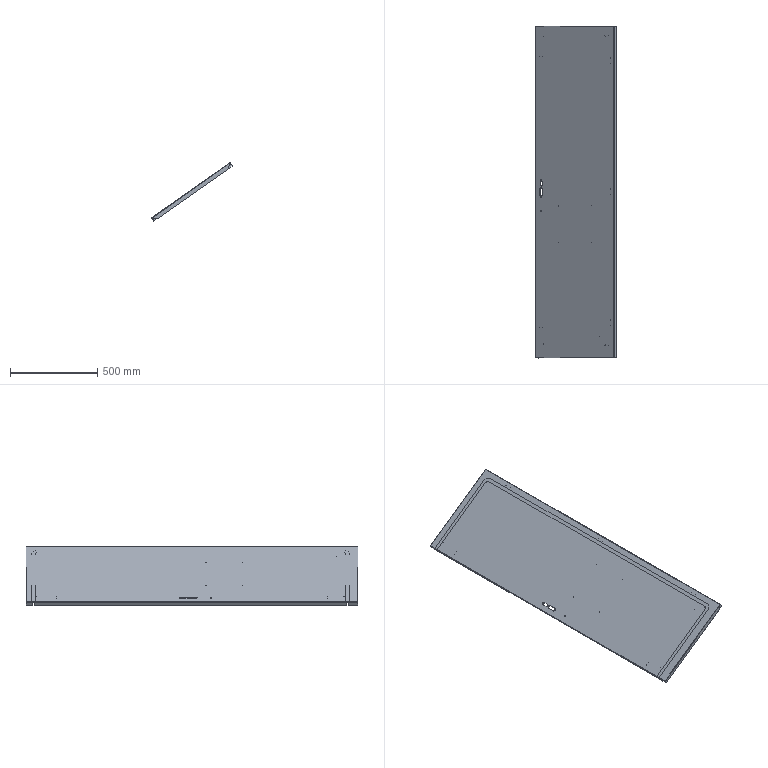Component | SolidWorks | FrontDoorLockHoleWeld-2_FrontDoorLockHole-1 | 1 solid | 169 faces | volume 1986258 mm3 | plane 98 | cylinder 67 | spline 4 | commonest cylinder face diameters 0.5 x38 3.2 x8 0.2 x8 8.5 x5 10 x4 70 x2 30 x2